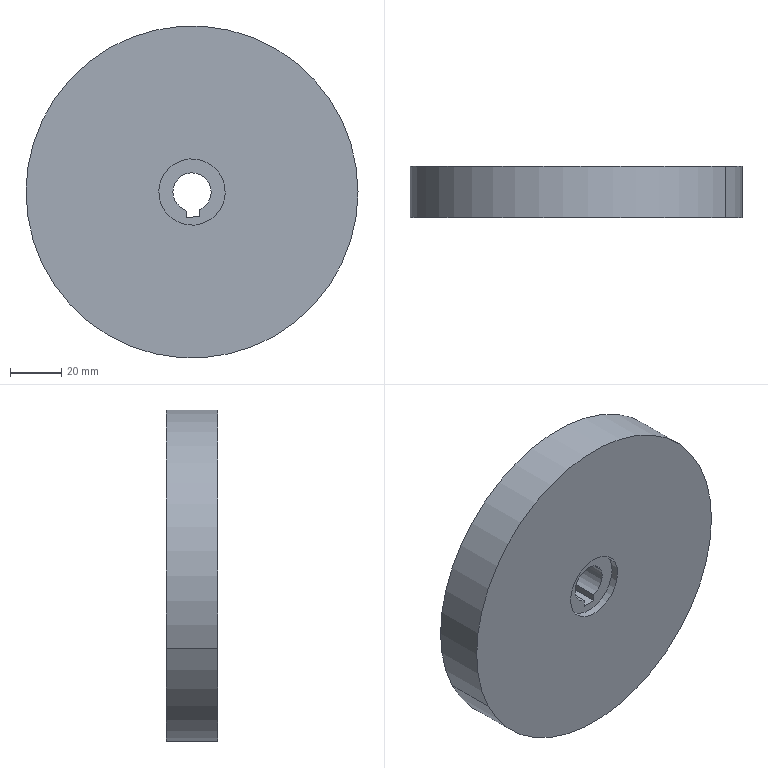Component | SolidWorks | ColumnRotationCylinderFlangePlate-1 | 1 solid | 13 faces | box 130 x 20 x 130 mm | volume 260651 mm3 | cylinder 7 | plane 6 | commonest cylinder face diameters 15 x3 26 x2 130 x2
build123d program:
from build123d import *

# Parameters (mm, degrees)
SKETCH1_2_R                       = 65
SKETCH1_2_R_2                     = 7.5
BOSS_EXTRUDE1_DEPTH               = 20
SKETCH1_R                         = 13
SHOULDER_RELIEF_COUNTERSINK_DEPTH = 3
KEYWAY_DEPTH                      = 95.074


with BuildPart() as part:
    # Sketch1_2 → Boss-Extrude1 (new body)
    with BuildSketch(Plane(origin=(0, 0, 0), x_dir=(1, 0, 0), z_dir=(0, 1, 0))):
        with Locations(Location((0, 0, 0), (0, 0, 270))):
            Circle(SKETCH1_2_R)
        with Locations(Location((0, 0, 0), (0, 0, 270))):
            Circle(SKETCH1_2_R_2, mode=Mode.SUBTRACT)
    extrude(amount=BOSS_EXTRUDE1_DEPTH)

    # Sketch1 → Shoulder Relief Countersink (cut)
    with BuildSketch(Plane.XZ):
        with Locations(Location((0.0012, -0.0015, 0), (0, 0, 270))):
            Circle(SKETCH1_R)
    extrude(amount=-SHOULDER_RELIEF_COUNTERSINK_DEPTH, mode=Mode.SUBTRACT)

    # Sketch2 → Keyway (cut, through all)
    with BuildSketch(Plane.XZ):
        Polygon((3.529, -4.396), (7.922, -6.331), (10.018, -1.572), (5.625, 0.3627), align=None)
    extrude(amount=-KEYWAY_DEPTH, mode=Mode.SUBTRACT)


solid = part.part

# Placed as in the assembly
solid = solid.moved(Location((-87.309, 188.019, 566.392), (0, 64.229, 0)))
STEP:
#1=COLOUR_RGB('',0.7922,0.8196,0.9333);
#2=FILL_AREA_STYLE_COLOUR('',#1);
#3=FILL_AREA_STYLE('',(#2));
#4=SURFACE_STYLE_FILL_AREA(#3);
#5=SURFACE_SIDE_STYLE('',(#4));
#6=SURFACE_STYLE_USAGE(.BOTH.,#5);
#7=PRESENTATION_STYLE_ASSIGNMENT((#6));
#8=CARTESIAN_POINT('',(-2.976,7.52,22.521));
#9=VERTEX_POINT('',#8);
#10=CARTESIAN_POINT('',(-3.898,7.52,22.076));
#11=VERTEX_POINT('',#10);
#12=CARTESIAN_POINT('',(-3.437,7.52,22.299));
#13=DIRECTION('',(0.,-1.,0.));
#14=DIRECTION('',(-0.9005,0.,-0.4348));
#15=AXIS2_PLACEMENT_3D('',#12,#13,#14);
#16=CIRCLE('',#15,0.5118);
#17=EDGE_CURVE('',#9,#11,#16,.T.);
#18=ORIENTED_EDGE('',*,*,#17,.F.);
#19=CARTESIAN_POINT('',(-2.976,7.402,22.521));
#20=VERTEX_POINT('',#19);
#21=CARTESIAN_POINT('',(-2.976,7.52,22.521));
#22=DIRECTION('',(0.,-1.,0.));
#23=VECTOR('',#22,39.37);
#24=LINE('',#21,#23);
#25=EDGE_CURVE('',#9,#20,#24,.T.);
#26=ORIENTED_EDGE('',*,*,#25,.T.);
#27=CARTESIAN_POINT('',(-3.898,7.402,22.076));
#28=VERTEX_POINT('',#27);
#29=CARTESIAN_POINT('',(-3.437,7.402,22.299));
#30=DIRECTION('',(0.,-1.,0.));
#31=DIRECTION('',(-0.9005,0.,-0.4348));
#32=AXIS2_PLACEMENT_3D('',#29,#30,#31);
#33=CIRCLE('',#32,0.5118);
#34=EDGE_CURVE('',#20,#28,#33,.T.);
#35=ORIENTED_EDGE('',*,*,#34,.T.);
#36=CARTESIAN_POINT('',(-3.898,7.52,22.076));
#37=DIRECTION('',(0.,-1.,0.));
#38=VECTOR('',#37,39.37);
#39=LINE('',#36,#38);
#40=EDGE_CURVE('',#11,#28,#39,.T.);
#41=ORIENTED_EDGE('',*,*,#40,.F.);
#42=EDGE_LOOP('',(#18,#26,#35,#41));
#43=FACE_OUTER_BOUND('',#42,.T.);
#44=CARTESIAN_POINT('',(-3.437,7.52,22.299));
#45=DIRECTION('',(0.,-1.,0.));
#46=DIRECTION('',(-0.9005,0.,-0.4348));
#47=AXIS2_PLACEMENT_3D('',#44,#45,#46);
#48=CYLINDRICAL_SURFACE('',#47,0.5118);
#49=ADVANCED_FACE('',(#43),#48,.F.);
#50=CARTESIAN_POINT('',(-1.133,8.19,23.412));
#51=VERTEX_POINT('',#50);
#52=CARTESIAN_POINT('',(-5.742,8.19,21.186));
#53=VERTEX_POINT('',#52);
#54=CARTESIAN_POINT('',(-3.437,8.19,22.299));
#55=DIRECTION('',(0.,1.,0.));
#56=DIRECTION('',(0.9005,0.,0.4348));
#57=AXIS2_PLACEMENT_3D('',#54,#55,#56);
#58=CIRCLE('',#57,2.559);
#59=EDGE_CURVE('',#51,#53,#58,.T.);
#60=ORIENTED_EDGE('',*,*,#59,.F.);
#61=CARTESIAN_POINT('',(-1.133,7.402,23.412));
#62=VERTEX_POINT('',#61);
#63=CARTESIAN_POINT('',(-1.133,8.19,23.412));
#64=DIRECTION('',(0.,-1.,0.));
#65=VECTOR('',#64,39.37);
#66=LINE('',#63,#65);
#67=EDGE_CURVE('',#51,#62,#66,.T.);
#68=ORIENTED_EDGE('',*,*,#67,.T.);
#69=CARTESIAN_POINT('',(-5.742,7.402,21.186));
#70=VERTEX_POINT('',#69);
#71=CARTESIAN_POINT('',(-3.437,7.402,22.299));
#72=DIRECTION('',(0.,1.,0.));
#73=DIRECTION('',(0.9005,0.,0.4348));
#74=AXIS2_PLACEMENT_3D('',#71,#72,#73);
#75=CIRCLE('',#74,2.559);
#76=EDGE_CURVE('',#62,#70,#75,.T.);
#77=ORIENTED_EDGE('',*,*,#76,.T.);
#78=CARTESIAN_POINT('',(-5.742,8.19,21.186));
#79=DIRECTION('',(0.,-1.,0.));
#80=VECTOR('',#79,39.37);
#81=LINE('',#78,#80);
#82=EDGE_CURVE('',#53,#70,#81,.T.);
#83=ORIENTED_EDGE('',*,*,#82,.F.);
#84=EDGE_LOOP('',(#60,#68,#77,#83));
#85=FACE_OUTER_BOUND('',#84,.T.);
#86=CARTESIAN_POINT('',(-3.437,8.19,22.299));
#87=DIRECTION('',(0.,-1.,0.));
#88=DIRECTION('',(-0.9005,0.,-0.4348));
#89=AXIS2_PLACEMENT_3D('',#86,#87,#88);
#90=CYLINDRICAL_SURFACE('',#89,2.559);
#91=ADVANCED_FACE('',(#85),#90,.T.);
#92=CARTESIAN_POINT('',(-3.703,8.19,22.171));
#93=VERTEX_POINT('',#92);
#94=CARTESIAN_POINT('',(-3.171,8.19,22.427));
#95=VERTEX_POINT('',#94);
#96=CARTESIAN_POINT('',(-3.437,8.19,22.299));
#97=DIRECTION('',(0.,1.,0.));
#98=DIRECTION('',(0.9005,0.,0.4348));
#99=AXIS2_PLACEMENT_3D('',#96,#97,#98);
#100=CIRCLE('',#99,0.2953);
#101=EDGE_CURVE('',#93,#95,#100,.T.);
#102=ORIENTED_EDGE('',*,*,#101,.T.);
#103=CARTESIAN_POINT('',(-3.171,7.52,22.427));
#104=VERTEX_POINT('',#103);
#105=CARTESIAN_POINT('',(-3.171,8.19,22.427));
#106=DIRECTION('',(0.,-1.,0.));
#107=VECTOR('',#106,39.37);
#108=LINE('',#105,#107);
#109=EDGE_CURVE('',#95,#104,#108,.T.);
#110=ORIENTED_EDGE('',*,*,#109,.T.);
#111=CARTESIAN_POINT('',(-3.703,7.52,22.171));
#112=VERTEX_POINT('',#111);
#113=CARTESIAN_POINT('',(-3.437,7.52,22.299));
#114=DIRECTION('',(0.,-1.,0.));
#115=DIRECTION('',(-0.9005,0.,-0.4348));
#116=AXIS2_PLACEMENT_3D('',#113,#114,#115);
#117=CIRCLE('',#116,0.2953);
#118=EDGE_CURVE('',#104,#112,#117,.T.);
#119=ORIENTED_EDGE('',*,*,#118,.T.);
#120=CARTESIAN_POINT('',(-3.703,8.19,22.171));
#121=DIRECTION('',(0.,-1.,0.));
#122=VECTOR('',#121,39.37);
#123=LINE('',#120,#122);
#124=EDGE_CURVE('',#93,#112,#123,.T.);
#125=ORIENTED_EDGE('',*,*,#124,.F.);
#126=EDGE_LOOP('',(#102,#110,#119,#125));
#127=FACE_OUTER_BOUND('',#126,.T.);
#128=CARTESIAN_POINT('',(-3.437,8.19,22.299));
#129=DIRECTION('',(0.,-1.,0.));
#130=DIRECTION('',(-0.9005,0.,-0.4348));
#131=AXIS2_PLACEMENT_3D('',#128,#129,#130);
#132=CYLINDRICAL_SURFACE('',#131,0.2953);
#133=ADVANCED_FACE('',(#127),#132,.F.);
#134=CARTESIAN_POINT('',(-3.53,8.19,22.019));
#135=VERTEX_POINT('',#134);
#136=CARTESIAN_POINT('',(-3.437,8.19,22.299));
#137=DIRECTION('',(0.,1.,0.));
#138=DIRECTION('',(0.9005,0.,0.4348));
#139=AXIS2_PLACEMENT_3D('',#136,#137,#138);
#140=CIRCLE('',#139,0.2953);
#141=EDGE_CURVE('',#135,#93,#140,.T.);
#142=ORIENTED_EDGE('',*,*,#141,.T.);
#143=ORIENTED_EDGE('',*,*,#124,.T.);
#144=CARTESIAN_POINT('',(-3.53,7.52,22.019));
#145=VERTEX_POINT('',#144);
#146=CARTESIAN_POINT('',(-3.437,7.52,22.299));
#147=DIRECTION('',(0.,-1.,0.));
#148=DIRECTION('',(-0.9005,0.,-0.4348));
#149=AXIS2_PLACEMENT_3D('',#146,#147,#148);
#150=CIRCLE('',#149,0.2953);
#151=EDGE_CURVE('',#112,#145,#150,.T.);
#152=ORIENTED_EDGE('',*,*,#151,.T.);
#153=CARTESIAN_POINT('',(-3.53,8.19,22.019));
#154=DIRECTION('',(0.,-1.,0.));
#155=VECTOR('',#154,39.37);
#156=LINE('',#153,#155);
#157=EDGE_CURVE('',#135,#145,#156,.T.);
#158=ORIENTED_EDGE('',*,*,#157,.F.);
#159=EDGE_LOOP('',(#142,#143,#152,#158));
#160=FACE_OUTER_BOUND('',#159,.T.);
#161=CARTESIAN_POINT('',(-3.437,8.19,22.299));
#162=DIRECTION('',(0.,-1.,0.));
#163=DIRECTION('',(-0.9005,0.,-0.4348));
#164=AXIS2_PLACEMENT_3D('',#161,#162,#163);
#165=CYLINDRICAL_SURFACE('',#164,0.2953);
#166=ADVANCED_FACE('',(#160),#165,.F.);
#167=CARTESIAN_POINT('',(-3.437,8.19,22.299));
#168=DIRECTION('',(0.,1.,0.));
#169=DIRECTION('',(0.9005,0.,0.4348));
#170=AXIS2_PLACEMENT_3D('',#167,#168,#169);
#171=CIRCLE('',#170,2.559);
#172=EDGE_CURVE('',#53,#51,#171,.T.);
#173=ORIENTED_EDGE('',*,*,#172,.T.);
#174=ORIENTED_EDGE('',*,*,#59,.T.);
#175=EDGE_LOOP('',(#173,#174));
#176=FACE_OUTER_BOUND('',#175,.T.);
#177=CARTESIAN_POINT('',(-3.526,8.19,21.91));
#178=VERTEX_POINT('',#177);
#179=CARTESIAN_POINT('',(-3.322,8.19,21.917));
#180=VERTEX_POINT('',#179);
#181=CARTESIAN_POINT('',(-3.526,8.19,21.91));
#182=DIRECTION('',(0.9994,0.,0.03494));
#183=VECTOR('',#182,39.37);
#184=LINE('',#181,#183);
#185=EDGE_CURVE('',#178,#180,#184,.T.);
#186=ORIENTED_EDGE('',*,*,#185,.T.);
#187=CARTESIAN_POINT('',(-3.325,8.19,22.026));
#188=VERTEX_POINT('',#187);
#189=CARTESIAN_POINT('',(-3.322,8.19,21.917));
#190=DIRECTION('',(-0.03494,0.,0.9994));
#191=VECTOR('',#190,39.37);
#192=LINE('',#189,#191);
#193=EDGE_CURVE('',#180,#188,#192,.T.);
#194=ORIENTED_EDGE('',*,*,#193,.T.);
#195=CARTESIAN_POINT('',(-3.437,8.19,22.299));
#196=DIRECTION('',(0.,1.,0.));
#197=DIRECTION('',(0.9005,0.,0.4348));
#198=AXIS2_PLACEMENT_3D('',#195,#196,#197);
#199=CIRCLE('',#198,0.2953);
#200=EDGE_CURVE('',#95,#188,#199,.T.);
#201=ORIENTED_EDGE('',*,*,#200,.F.);
#202=ORIENTED_EDGE('',*,*,#101,.F.);
#203=ORIENTED_EDGE('',*,*,#141,.F.);
#204=CARTESIAN_POINT('',(-3.533,8.19,22.099));
#205=DIRECTION('',(0.03494,0.,-0.9994));
#206=VECTOR('',#205,39.37);
#207=LINE('',#204,#206);
#208=EDGE_CURVE('',#135,#178,#207,.T.);
#209=ORIENTED_EDGE('',*,*,#208,.T.);
#210=EDGE_LOOP('',(#186,#194,#201,#202,#203,#209));
#211=FACE_BOUND('',#210,.T.);
#212=CARTESIAN_POINT('',(-3.437,8.19,22.299));
#213=DIRECTION('',(0.,1.,0.));
#214=DIRECTION('',(0.9005,0.,0.4348));
#215=AXIS2_PLACEMENT_3D('',#212,#213,#214);
#216=PLANE('',#215);
#217=ADVANCED_FACE('',(#176,#211),#216,.T.);
#218=ORIENTED_EDGE('',*,*,#109,.F.);
#219=ORIENTED_EDGE('',*,*,#200,.T.);
#220=CARTESIAN_POINT('',(-3.325,7.52,22.026));
#221=VERTEX_POINT('',#220);
#222=CARTESIAN_POINT('',(-3.325,8.19,22.026));
#223=DIRECTION('',(0.,1.,0.));
#224=VECTOR('',#223,39.37);
#225=LINE('',#222,#224);
#226=EDGE_CURVE('',#221,#188,#225,.T.);
#227=ORIENTED_EDGE('',*,*,#226,.F.);
#228=CARTESIAN_POINT('',(-3.437,7.52,22.299));
#229=DIRECTION('',(0.,-1.,0.));
#230=DIRECTION('',(-0.9005,0.,-0.4348));
#231=AXIS2_PLACEMENT_3D('',#228,#229,#230);
#232=CIRCLE('',#231,0.2953);
#233=EDGE_CURVE('',#221,#104,#232,.T.);
#234=ORIENTED_EDGE('',*,*,#233,.T.);
#235=EDGE_LOOP('',(#218,#219,#227,#234));
#236=FACE_OUTER_BOUND('',#235,.T.);
#237=CARTESIAN_POINT('',(-3.437,8.19,22.299));
#238=DIRECTION('',(0.,-1.,0.));
#239=DIRECTION('',(-0.9005,0.,-0.4348));
#240=AXIS2_PLACEMENT_3D('',#237,#238,#239);
#241=CYLINDRICAL_SURFACE('',#240,0.2953);
#242=ADVANCED_FACE('',(#236),#241,.F.);
#243=CARTESIAN_POINT('',(-3.437,7.402,22.299));
#244=DIRECTION('',(0.,-1.,0.));
#245=DIRECTION('',(-0.9005,0.,-0.4348));
#246=AXIS2_PLACEMENT_3D('',#243,#244,#245);
#247=CIRCLE('',#246,0.5118);
#248=EDGE_CURVE('',#28,#20,#247,.T.);
#249=ORIENTED_EDGE('',*,*,#248,.F.);
#250=ORIENTED_EDGE('',*,*,#34,.F.);
#251=EDGE_LOOP('',(#249,#250));
#252=FACE_BOUND('',#251,.T.);
#253=CARTESIAN_POINT('',(-3.437,7.402,22.299));
#254=DIRECTION('',(0.,1.,0.));
#255=DIRECTION('',(0.9005,0.,0.4348));
#256=AXIS2_PLACEMENT_3D('',#253,#254,#255);
#257=CIRCLE('',#256,2.559);
#258=EDGE_CURVE('',#70,#62,#257,.T.);
#259=ORIENTED_EDGE('',*,*,#258,.F.);
#260=ORIENTED_EDGE('',*,*,#76,.F.);
#261=EDGE_LOOP('',(#259,#260));
#262=FACE_OUTER_BOUND('',#261,.T.);
#263=CARTESIAN_POINT('',(-3.437,7.402,22.299));
#264=DIRECTION('',(0.,1.,0.));
#265=DIRECTION('',(0.9005,0.,0.4348));
#266=AXIS2_PLACEMENT_3D('',#263,#264,#265);
#267=PLANE('',#266);
#268=ADVANCED_FACE('',(#252,#262),#267,.F.);
#269=ORIENTED_EDGE('',*,*,#67,.F.);
#270=ORIENTED_EDGE('',*,*,#172,.F.);
#271=ORIENTED_EDGE('',*,*,#82,.T.);
#272=ORIENTED_EDGE('',*,*,#258,.T.);
#273=EDGE_LOOP('',(#269,#270,#271,#272));
#274=FACE_OUTER_BOUND('',#273,.T.);
#275=CARTESIAN_POINT('',(-3.437,8.19,22.299));
#276=DIRECTION('',(0.,-1.,0.));
#277=DIRECTION('',(-0.9005,0.,-0.4348));
#278=AXIS2_PLACEMENT_3D('',#275,#276,#277);
#279=CYLINDRICAL_SURFACE('',#278,2.559);
#280=ADVANCED_FACE('',(#274),#279,.T.);
#281=ORIENTED_EDGE('',*,*,#25,.F.);
#282=CARTESIAN_POINT('',(-3.437,7.52,22.299));
#283=DIRECTION('',(0.,-1.,0.));
#284=DIRECTION('',(-0.9005,0.,-0.4348));
#285=AXIS2_PLACEMENT_3D('',#282,#283,#284);
#286=CIRCLE('',#285,0.5118);
#287=EDGE_CURVE('',#11,#9,#286,.T.);
#288=ORIENTED_EDGE('',*,*,#287,.F.);
#289=ORIENTED_EDGE('',*,*,#40,.T.);
#290=ORIENTED_EDGE('',*,*,#248,.T.);
#291=EDGE_LOOP('',(#281,#288,#289,#290));
#292=FACE_OUTER_BOUND('',#291,.T.);
#293=CARTESIAN_POINT('',(-3.437,7.52,22.299));
#294=DIRECTION('',(0.,-1.,0.));
#295=DIRECTION('',(-0.9005,0.,-0.4348));
#296=AXIS2_PLACEMENT_3D('',#293,#294,#295);
#297=CYLINDRICAL_SURFACE('',#296,0.5118);
#298=ADVANCED_FACE('',(#292),#297,.F.);
#299=CARTESIAN_POINT('',(-3.322,7.52,21.917));
#300=VERTEX_POINT('',#299);
#301=CARTESIAN_POINT('',(-3.335,7.52,22.302));
#302=DIRECTION('',(-0.03494,0.,0.9994));
#303=VECTOR('',#302,39.37);
#304=LINE('',#301,#303);
#305=EDGE_CURVE('',#300,#221,#304,.T.);
#306=ORIENTED_EDGE('',*,*,#305,.F.);
#307=CARTESIAN_POINT('',(-3.526,7.52,21.91));
#308=VERTEX_POINT('',#307);
#309=CARTESIAN_POINT('',(-3.424,7.52,21.913));
#310=DIRECTION('',(0.9994,0.,0.03494));
#311=VECTOR('',#310,39.37);
#312=LINE('',#309,#311);
#313=EDGE_CURVE('',#308,#300,#312,.T.);
#314=ORIENTED_EDGE('',*,*,#313,.F.);
#315=CARTESIAN_POINT('',(-3.54,7.52,22.295));
#316=DIRECTION('',(0.03494,0.,-0.9994));
#317=VECTOR('',#316,39.37);
#318=LINE('',#315,#317);
#319=EDGE_CURVE('',#145,#308,#318,.T.);
#320=ORIENTED_EDGE('',*,*,#319,.F.);
#321=ORIENTED_EDGE('',*,*,#151,.F.);
#322=ORIENTED_EDGE('',*,*,#118,.F.);
#323=ORIENTED_EDGE('',*,*,#233,.F.);
#324=EDGE_LOOP('',(#306,#314,#320,#321,#322,#323));
#325=FACE_BOUND('',#324,.T.);
#326=ORIENTED_EDGE('',*,*,#287,.T.);
#327=ORIENTED_EDGE('',*,*,#17,.T.);
#328=EDGE_LOOP('',(#326,#327));
#329=FACE_OUTER_BOUND('',#328,.T.);
#330=CARTESIAN_POINT('',(-3.437,7.52,22.299));
#331=DIRECTION('',(0.,-1.,0.));
#332=DIRECTION('',(-0.9005,0.,-0.4348));
#333=AXIS2_PLACEMENT_3D('',#330,#331,#332);
#334=PLANE('',#333);
#335=ADVANCED_FACE('',(#325,#329),#334,.T.);
#336=ORIENTED_EDGE('',*,*,#226,.T.);
#337=ORIENTED_EDGE('',*,*,#193,.F.);
#338=CARTESIAN_POINT('',(-3.322,8.19,21.917));
#339=DIRECTION('',(0.,-1.,0.));
#340=VECTOR('',#339,39.37);
#341=LINE('',#338,#340);
#342=EDGE_CURVE('',#180,#300,#341,.T.);
#343=ORIENTED_EDGE('',*,*,#342,.T.);
#344=ORIENTED_EDGE('',*,*,#305,.T.);
#345=EDGE_LOOP('',(#336,#337,#343,#344));
#346=FACE_OUTER_BOUND('',#345,.T.);
#347=CARTESIAN_POINT('',(-3.322,8.19,21.917));
#348=DIRECTION('',(0.9994,0.,0.03494));
#349=DIRECTION('',(0.03494,0.,-0.9994));
#350=AXIS2_PLACEMENT_3D('',#347,#348,#349);
#351=PLANE('',#350);
#352=ADVANCED_FACE('',(#346),#351,.F.);
#353=ORIENTED_EDGE('',*,*,#313,.T.);
#354=ORIENTED_EDGE('',*,*,#342,.F.);
#355=ORIENTED_EDGE('',*,*,#185,.F.);
#356=CARTESIAN_POINT('',(-3.526,8.19,21.91));
#357=DIRECTION('',(0.,-1.,0.));
#358=VECTOR('',#357,39.37);
#359=LINE('',#356,#358);
#360=EDGE_CURVE('',#178,#308,#359,.T.);
#361=ORIENTED_EDGE('',*,*,#360,.T.);
#362=EDGE_LOOP('',(#353,#354,#355,#361));
#363=FACE_OUTER_BOUND('',#362,.T.);
#364=CARTESIAN_POINT('',(-3.526,8.19,21.91));
#365=DIRECTION('',(0.03494,0.,-0.9994));
#366=DIRECTION('',(-0.9994,0.,-0.03494));
#367=AXIS2_PLACEMENT_3D('',#364,#365,#366);
#368=PLANE('',#367);
#369=ADVANCED_FACE('',(#363),#368,.F.);
#370=ORIENTED_EDGE('',*,*,#157,.T.);
#371=ORIENTED_EDGE('',*,*,#319,.T.);
#372=ORIENTED_EDGE('',*,*,#360,.F.);
#373=ORIENTED_EDGE('',*,*,#208,.F.);
#374=EDGE_LOOP('',(#370,#371,#372,#373));
#375=FACE_OUTER_BOUND('',#374,.T.);
#376=CARTESIAN_POINT('',(-3.533,8.19,22.099));
#377=DIRECTION('',(-0.9994,0.,-0.03494));
#378=DIRECTION('',(-0.03494,0.,0.9994));
#379=AXIS2_PLACEMENT_3D('',#376,#377,#378);
#380=PLANE('',#379);
#381=ADVANCED_FACE('',(#375),#380,.F.);
#382=CLOSED_SHELL('',(#49,#91,#133,#166,#217,#242,#268,#280,#298,#335,#352,#369,#381));
#383=MANIFOLD_SOLID_BREP('',#382);
#384=STYLED_ITEM('',(#7),#383);
#385=PRESENTATION_LAYER_ASSIGNMENT('','',(#384));
#386=(LENGTH_UNIT()NAMED_UNIT(*)SI_UNIT($,.METRE.));
#387=LENGTH_MEASURE_WITH_UNIT(LENGTH_MEASURE(0.0254),#386);
#388=DIMENSIONAL_EXPONENTS(1.,0.,0.,0.,0.,0.,0.);
#389=(CONVERSION_BASED_UNIT('',#387)LENGTH_UNIT()NAMED_UNIT(#388));
#390=UNCERTAINTY_MEASURE_WITH_UNIT(LENGTH_MEASURE(0.00001),#389,'','');
#391=(NAMED_UNIT(*)PLANE_ANGLE_UNIT()SI_UNIT($,.RADIAN.));
#392=(NAMED_UNIT(*)SI_UNIT($,.STERADIAN.)SOLID_ANGLE_UNIT());
#393=(GEOMETRIC_REPRESENTATION_CONTEXT(3)GLOBAL_UNCERTAINTY_ASSIGNED_CONTEXT((#390))GLOBAL_UNIT_ASSIGNED_CONTEXT((#389,#391,#392))REPRESENTATION_CONTEXT('',''));
#394=MECHANICAL_DESIGN_GEOMETRIC_PRESENTATION_REPRESENTATION('',(#384),#393);
#395=CARTESIAN_POINT('',(0.,0.,0.));
#396=DIRECTION('',(0.,0.,1.));
#397=DIRECTION('',(1.,0.,0.));
#398=AXIS2_PLACEMENT_3D('',#395,#396,#397);
#399=(LENGTH_UNIT()NAMED_UNIT(*)SI_UNIT($,.METRE.));
#400=LENGTH_MEASURE_WITH_UNIT(LENGTH_MEASURE(0.0254),#399);
#401=DIMENSIONAL_EXPONENTS(1.,0.,0.,0.,0.,0.,0.);
#402=(CONVERSION_BASED_UNIT('',#400)LENGTH_UNIT()NAMED_UNIT(#401));
#403=UNCERTAINTY_MEASURE_WITH_UNIT(LENGTH_MEASURE(0.00001),#402,'','');
#404=(NAMED_UNIT(*)PLANE_ANGLE_UNIT()SI_UNIT($,.RADIAN.));
#405=(NAMED_UNIT(*)SI_UNIT($,.STERADIAN.)SOLID_ANGLE_UNIT());
#406=(GEOMETRIC_REPRESENTATION_CONTEXT(3)GLOBAL_UNCERTAINTY_ASSIGNED_CONTEXT((#403))GLOBAL_UNIT_ASSIGNED_CONTEXT((#402,#404,#405))REPRESENTATION_CONTEXT('',''));
#407=ADVANCED_BREP_SHAPE_REPRESENTATION('',(#383,#398),#406);